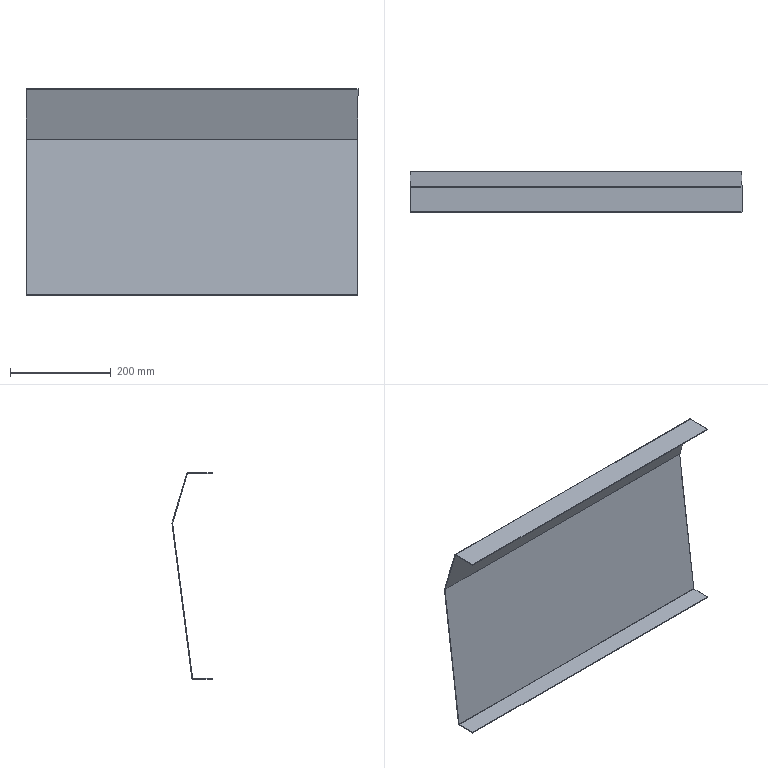Component | SolidWorks | RainproofTopCover-1 | 1 solid | 30 faces | box 660 x 79.97 x 410 mm | volume 498730 mm3 | plane 24 | cylinder 6 | commonest cylinder face diameters 3.2 x3 0.2 x3
STEP:
#1=COLOUR_RGB('',0.7922,0.8196,0.9333);
#2=FILL_AREA_STYLE_COLOUR('',#1);
#3=FILL_AREA_STYLE('',(#2));
#4=SURFACE_STYLE_FILL_AREA(#3);
#5=SURFACE_SIDE_STYLE('',(#4));
#6=SURFACE_STYLE_USAGE(.BOTH.,#5);
#7=PRESENTATION_STYLE_ASSIGNMENT((#6));
#8=CARTESIAN_POINT('',(-14.739,15.415,23.545));
#9=VERTEX_POINT('',#8);
#10=CARTESIAN_POINT('',(-14.739,15.357,23.552));
#11=VERTEX_POINT('',#10);
#12=CARTESIAN_POINT('',(-14.739,15.415,23.545));
#13=DIRECTION('',(0.,-0.9918,0.128));
#14=VECTOR('',#13,39.37);
#15=LINE('',#12,#14);
#16=EDGE_CURVE('',#9,#11,#15,.T.);
#17=ORIENTED_EDGE('',*,*,#16,.F.);
#18=CARTESIAN_POINT('',(-14.739,15.353,23.49));
#19=VERTEX_POINT('',#18);
#20=CARTESIAN_POINT('',(-14.739,15.353,23.553));
#21=DIRECTION('',(1.,0.,-0.));
#22=DIRECTION('',(0.,0.,1.));
#23=AXIS2_PLACEMENT_3D('',#20,#21,#22);
#24=CIRCLE('',#23,0.06299);
#25=EDGE_CURVE('',#19,#9,#24,.T.);
#26=ORIENTED_EDGE('',*,*,#25,.F.);
#27=CARTESIAN_POINT('',(-14.739,15.353,23.549));
#28=VERTEX_POINT('',#27);
#29=CARTESIAN_POINT('',(-14.739,15.353,23.549));
#30=DIRECTION('',(-0.,0.,-1.));
#31=VECTOR('',#30,39.37);
#32=LINE('',#29,#31);
#33=EDGE_CURVE('',#28,#19,#32,.T.);
#34=ORIENTED_EDGE('',*,*,#33,.F.);
#35=CARTESIAN_POINT('',(-14.739,15.353,23.553));
#36=DIRECTION('',(1.,0.,-0.));
#37=DIRECTION('',(0.,0.,1.));
#38=AXIS2_PLACEMENT_3D('',#35,#36,#37);
#39=CIRCLE('',#38,0.003937);
#40=EDGE_CURVE('',#28,#11,#39,.T.);
#41=ORIENTED_EDGE('',*,*,#40,.T.);
#42=EDGE_LOOP('',(#17,#26,#34,#41));
#43=FACE_OUTER_BOUND('',#42,.T.);
#44=CARTESIAN_POINT('',(-14.739,15.415,23.545));
#45=DIRECTION('',(-1.,-0.,0.));
#46=DIRECTION('',(0.,-0.,1.));
#47=AXIS2_PLACEMENT_3D('',#44,#45,#46);
#48=PLANE('',#47);
#49=ADVANCED_FACE('',(#43),#48,.T.);
#50=CARTESIAN_POINT('',(-14.739,16.981,35.681));
#51=VERTEX_POINT('',#50);
#52=CARTESIAN_POINT('',(-14.739,15.408,23.49));
#53=DIRECTION('',(0.,0.128,0.9918));
#54=VECTOR('',#53,39.37);
#55=LINE('',#52,#54);
#56=EDGE_CURVE('',#9,#51,#55,.T.);
#57=ORIENTED_EDGE('',*,*,#56,.F.);
#58=ORIENTED_EDGE('',*,*,#16,.T.);
#59=CARTESIAN_POINT('',(-14.739,16.923,35.689));
#60=VERTEX_POINT('',#59);
#61=CARTESIAN_POINT('',(-14.739,15.35,23.497));
#62=DIRECTION('',(0.,0.128,0.9918));
#63=VECTOR('',#62,39.37);
#64=LINE('',#61,#63);
#65=EDGE_CURVE('',#11,#60,#64,.T.);
#66=ORIENTED_EDGE('',*,*,#65,.T.);
#67=CARTESIAN_POINT('',(-14.739,16.923,35.689));
#68=DIRECTION('',(-0.,0.9918,-0.128));
#69=VECTOR('',#68,39.37);
#70=LINE('',#67,#69);
#71=EDGE_CURVE('',#60,#51,#70,.T.);
#72=ORIENTED_EDGE('',*,*,#71,.T.);
#73=EDGE_LOOP('',(#57,#58,#66,#72));
#74=FACE_OUTER_BOUND('',#73,.T.);
#75=CARTESIAN_POINT('',(-14.739,15.353,23.549));
#76=DIRECTION('',(-1.,-0.,0.));
#77=DIRECTION('',(0.,-0.,1.));
#78=AXIS2_PLACEMENT_3D('',#75,#76,#77);
#79=PLANE('',#78);
#80=ADVANCED_FACE('',(#74),#79,.T.);
#81=CARTESIAN_POINT('',(11.246,15.353,23.49));
#82=VERTEX_POINT('',#81);
#83=CARTESIAN_POINT('',(11.246,15.353,23.549));
#84=VERTEX_POINT('',#83);
#85=CARTESIAN_POINT('',(11.246,15.353,23.49));
#86=DIRECTION('',(0.,-0.,1.));
#87=VECTOR('',#86,39.37);
#88=LINE('',#85,#87);
#89=EDGE_CURVE('',#82,#84,#88,.T.);
#90=ORIENTED_EDGE('',*,*,#89,.F.);
#91=CARTESIAN_POINT('',(11.246,15.415,23.545));
#92=VERTEX_POINT('',#91);
#93=CARTESIAN_POINT('',(11.246,15.353,23.553));
#94=DIRECTION('',(1.,0.,-0.));
#95=DIRECTION('',(0.,0.,1.));
#96=AXIS2_PLACEMENT_3D('',#93,#94,#95);
#97=CIRCLE('',#96,0.06299);
#98=EDGE_CURVE('',#82,#92,#97,.T.);
#99=ORIENTED_EDGE('',*,*,#98,.T.);
#100=CARTESIAN_POINT('',(11.246,15.357,23.552));
#101=VERTEX_POINT('',#100);
#102=CARTESIAN_POINT('',(11.246,15.357,23.552));
#103=DIRECTION('',(-0.,0.9918,-0.128));
#104=VECTOR('',#103,39.37);
#105=LINE('',#102,#104);
#106=EDGE_CURVE('',#101,#92,#105,.T.);
#107=ORIENTED_EDGE('',*,*,#106,.F.);
#108=CARTESIAN_POINT('',(11.246,15.353,23.553));
#109=DIRECTION('',(1.,0.,-0.));
#110=DIRECTION('',(0.,0.,1.));
#111=AXIS2_PLACEMENT_3D('',#108,#109,#110);
#112=CIRCLE('',#111,0.003937);
#113=EDGE_CURVE('',#84,#101,#112,.T.);
#114=ORIENTED_EDGE('',*,*,#113,.F.);
#115=EDGE_LOOP('',(#90,#99,#107,#114));
#116=FACE_OUTER_BOUND('',#115,.T.);
#117=CARTESIAN_POINT('',(11.246,15.353,23.49));
#118=DIRECTION('',(1.,0.,-0.));
#119=DIRECTION('',(-0.,0.,-1.));
#120=AXIS2_PLACEMENT_3D('',#117,#118,#119);
#121=PLANE('',#120);
#122=ADVANCED_FACE('',(#116),#121,.T.);
#123=CARTESIAN_POINT('',(11.246,13.833,23.49));
#124=VERTEX_POINT('',#123);
#125=CARTESIAN_POINT('',(11.246,13.833,23.49));
#126=DIRECTION('',(0.,1.,0.));
#127=VECTOR('',#126,39.37);
#128=LINE('',#125,#127);
#129=EDGE_CURVE('',#124,#82,#128,.T.);
#130=ORIENTED_EDGE('',*,*,#129,.T.);
#131=ORIENTED_EDGE('',*,*,#89,.T.);
#132=CARTESIAN_POINT('',(11.246,13.833,23.549));
#133=VERTEX_POINT('',#132);
#134=CARTESIAN_POINT('',(11.246,13.833,23.549));
#135=DIRECTION('',(0.,1.,0.));
#136=VECTOR('',#135,39.37);
#137=LINE('',#134,#136);
#138=EDGE_CURVE('',#133,#84,#137,.T.);
#139=ORIENTED_EDGE('',*,*,#138,.F.);
#140=CARTESIAN_POINT('',(11.246,13.833,23.549));
#141=DIRECTION('',(-0.,0.,-1.));
#142=VECTOR('',#141,39.37);
#143=LINE('',#140,#142);
#144=EDGE_CURVE('',#133,#124,#143,.T.);
#145=ORIENTED_EDGE('',*,*,#144,.T.);
#146=EDGE_LOOP('',(#130,#131,#139,#145));
#147=FACE_OUTER_BOUND('',#146,.T.);
#148=CARTESIAN_POINT('',(11.246,15.357,23.552));
#149=DIRECTION('',(1.,0.,-0.));
#150=DIRECTION('',(-0.,0.,-1.));
#151=AXIS2_PLACEMENT_3D('',#148,#149,#150);
#152=PLANE('',#151);
#153=ADVANCED_FACE('',(#147),#152,.T.);
#154=CARTESIAN_POINT('',(-14.739,16.979,35.707));
#155=VERTEX_POINT('',#154);
#156=CARTESIAN_POINT('',(-14.739,16.923,35.69));
#157=VERTEX_POINT('',#156);
#158=CARTESIAN_POINT('',(-14.739,16.979,35.707));
#159=DIRECTION('',(-0.,-0.9578,-0.2873));
#160=VECTOR('',#159,39.37);
#161=LINE('',#158,#160);
#162=EDGE_CURVE('',#155,#157,#161,.T.);
#163=ORIENTED_EDGE('',*,*,#162,.F.);
#164=CARTESIAN_POINT('',(-14.739,16.919,35.689));
#165=DIRECTION('',(1.,0.,-0.));
#166=DIRECTION('',(0.,0.,1.));
#167=AXIS2_PLACEMENT_3D('',#164,#165,#166);
#168=CIRCLE('',#167,0.06299);
#169=EDGE_CURVE('',#51,#155,#168,.T.);
#170=ORIENTED_EDGE('',*,*,#169,.F.);
#171=ORIENTED_EDGE('',*,*,#71,.F.);
#172=CARTESIAN_POINT('',(-14.739,16.919,35.689));
#173=DIRECTION('',(1.,0.,-0.));
#174=DIRECTION('',(0.,0.,1.));
#175=AXIS2_PLACEMENT_3D('',#172,#173,#174);
#176=CIRCLE('',#175,0.003937);
#177=EDGE_CURVE('',#60,#157,#176,.T.);
#178=ORIENTED_EDGE('',*,*,#177,.T.);
#179=EDGE_LOOP('',(#163,#170,#171,#178));
#180=FACE_OUTER_BOUND('',#179,.T.);
#181=CARTESIAN_POINT('',(-14.739,16.979,35.707));
#182=DIRECTION('',(-1.,-0.,0.));
#183=DIRECTION('',(0.,-0.,1.));
#184=AXIS2_PLACEMENT_3D('',#181,#182,#183);
#185=PLANE('',#184);
#186=ADVANCED_FACE('',(#180),#185,.T.);
#187=CARTESIAN_POINT('',(-14.739,15.815,39.586));
#188=VERTEX_POINT('',#187);
#189=CARTESIAN_POINT('',(-14.739,16.983,35.694));
#190=DIRECTION('',(0.,-0.2873,0.9578));
#191=VECTOR('',#190,39.37);
#192=LINE('',#189,#191);
#193=EDGE_CURVE('',#155,#188,#192,.T.);
#194=ORIENTED_EDGE('',*,*,#193,.F.);
#195=ORIENTED_EDGE('',*,*,#162,.T.);
#196=CARTESIAN_POINT('',(-14.739,15.759,39.57));
#197=VERTEX_POINT('',#196);
#198=CARTESIAN_POINT('',(-14.739,16.926,35.677));
#199=DIRECTION('',(0.,-0.2873,0.9578));
#200=VECTOR('',#199,39.37);
#201=LINE('',#198,#200);
#202=EDGE_CURVE('',#157,#197,#201,.T.);
#203=ORIENTED_EDGE('',*,*,#202,.T.);
#204=CARTESIAN_POINT('',(-14.739,15.759,39.57));
#205=DIRECTION('',(0.,0.9578,0.2873));
#206=VECTOR('',#205,39.37);
#207=LINE('',#204,#206);
#208=EDGE_CURVE('',#197,#188,#207,.T.);
#209=ORIENTED_EDGE('',*,*,#208,.T.);
#210=EDGE_LOOP('',(#194,#195,#203,#209));
#211=FACE_OUTER_BOUND('',#210,.T.);
#212=CARTESIAN_POINT('',(-14.739,16.923,35.689));
#213=DIRECTION('',(-1.,-0.,0.));
#214=DIRECTION('',(0.,-0.,1.));
#215=AXIS2_PLACEMENT_3D('',#212,#213,#214);
#216=PLANE('',#215);
#217=ADVANCED_FACE('',(#211),#216,.T.);
#218=CARTESIAN_POINT('',(11.246,16.981,35.681));
#219=VERTEX_POINT('',#218);
#220=CARTESIAN_POINT('',(11.246,16.923,35.689));
#221=VERTEX_POINT('',#220);
#222=CARTESIAN_POINT('',(11.246,16.981,35.681));
#223=DIRECTION('',(0.,-0.9918,0.128));
#224=VECTOR('',#223,39.37);
#225=LINE('',#222,#224);
#226=EDGE_CURVE('',#219,#221,#225,.T.);
#227=ORIENTED_EDGE('',*,*,#226,.F.);
#228=CARTESIAN_POINT('',(11.246,16.979,35.707));
#229=VERTEX_POINT('',#228);
#230=CARTESIAN_POINT('',(11.246,16.919,35.689));
#231=DIRECTION('',(1.,0.,-0.));
#232=DIRECTION('',(0.,0.,1.));
#233=AXIS2_PLACEMENT_3D('',#230,#231,#232);
#234=CIRCLE('',#233,0.06299);
#235=EDGE_CURVE('',#219,#229,#234,.T.);
#236=ORIENTED_EDGE('',*,*,#235,.T.);
#237=CARTESIAN_POINT('',(11.246,16.923,35.69));
#238=VERTEX_POINT('',#237);
#239=CARTESIAN_POINT('',(11.246,16.923,35.69));
#240=DIRECTION('',(0.,0.9578,0.2873));
#241=VECTOR('',#240,39.37);
#242=LINE('',#239,#241);
#243=EDGE_CURVE('',#238,#229,#242,.T.);
#244=ORIENTED_EDGE('',*,*,#243,.F.);
#245=CARTESIAN_POINT('',(11.246,16.919,35.689));
#246=DIRECTION('',(1.,0.,-0.));
#247=DIRECTION('',(0.,0.,1.));
#248=AXIS2_PLACEMENT_3D('',#245,#246,#247);
#249=CIRCLE('',#248,0.003937);
#250=EDGE_CURVE('',#221,#238,#249,.T.);
#251=ORIENTED_EDGE('',*,*,#250,.F.);
#252=EDGE_LOOP('',(#227,#236,#244,#251));
#253=FACE_OUTER_BOUND('',#252,.T.);
#254=CARTESIAN_POINT('',(11.246,16.981,35.681));
#255=DIRECTION('',(1.,0.,-0.));
#256=DIRECTION('',(-0.,0.,-1.));
#257=AXIS2_PLACEMENT_3D('',#254,#255,#256);
#258=PLANE('',#257);
#259=ADVANCED_FACE('',(#253),#258,.T.);
#260=CARTESIAN_POINT('',(11.246,15.408,23.49));
#261=DIRECTION('',(0.,0.128,0.9918));
#262=VECTOR('',#261,39.37);
#263=LINE('',#260,#262);
#264=EDGE_CURVE('',#92,#219,#263,.T.);
#265=ORIENTED_EDGE('',*,*,#264,.T.);
#266=ORIENTED_EDGE('',*,*,#226,.T.);
#267=CARTESIAN_POINT('',(11.246,15.35,23.497));
#268=DIRECTION('',(0.,0.128,0.9918));
#269=VECTOR('',#268,39.37);
#270=LINE('',#267,#269);
#271=EDGE_CURVE('',#101,#221,#270,.T.);
#272=ORIENTED_EDGE('',*,*,#271,.F.);
#273=ORIENTED_EDGE('',*,*,#106,.T.);
#274=EDGE_LOOP('',(#265,#266,#272,#273));
#275=FACE_OUTER_BOUND('',#274,.T.);
#276=CARTESIAN_POINT('',(11.246,16.923,35.69));
#277=DIRECTION('',(1.,0.,-0.));
#278=DIRECTION('',(-0.,0.,-1.));
#279=AXIS2_PLACEMENT_3D('',#276,#277,#278);
#280=PLANE('',#279);
#281=ADVANCED_FACE('',(#275),#280,.T.);
#282=CARTESIAN_POINT('',(-14.739,15.755,39.631));
#283=VERTEX_POINT('',#282);
#284=CARTESIAN_POINT('',(-14.739,15.755,39.572));
#285=VERTEX_POINT('',#284);
#286=CARTESIAN_POINT('',(-14.739,15.755,39.631));
#287=DIRECTION('',(-0.,0.,-1.));
#288=VECTOR('',#287,39.37);
#289=LINE('',#286,#288);
#290=EDGE_CURVE('',#283,#285,#289,.T.);
#291=ORIENTED_EDGE('',*,*,#290,.F.);
#292=CARTESIAN_POINT('',(-14.739,15.755,39.568));
#293=DIRECTION('',(1.,0.,-0.));
#294=DIRECTION('',(0.,-0.,1.));
#295=AXIS2_PLACEMENT_3D('',#292,#293,#294);
#296=CIRCLE('',#295,0.06299);
#297=EDGE_CURVE('',#188,#283,#296,.T.);
#298=ORIENTED_EDGE('',*,*,#297,.F.);
#299=ORIENTED_EDGE('',*,*,#208,.F.);
#300=CARTESIAN_POINT('',(-14.739,15.755,39.568));
#301=DIRECTION('',(1.,0.,-0.));
#302=DIRECTION('',(0.,0.,1.));
#303=AXIS2_PLACEMENT_3D('',#300,#301,#302);
#304=CIRCLE('',#303,0.003937);
#305=EDGE_CURVE('',#197,#285,#304,.T.);
#306=ORIENTED_EDGE('',*,*,#305,.T.);
#307=EDGE_LOOP('',(#291,#298,#299,#306));
#308=FACE_OUTER_BOUND('',#307,.T.);
#309=CARTESIAN_POINT('',(-14.739,15.755,39.631));
#310=DIRECTION('',(-1.,-0.,0.));
#311=DIRECTION('',(0.,-0.,1.));
#312=AXIS2_PLACEMENT_3D('',#309,#310,#311);
#313=PLANE('',#312);
#314=ADVANCED_FACE('',(#308),#313,.T.);
#315=CARTESIAN_POINT('',(-14.739,13.833,39.631));
#316=VERTEX_POINT('',#315);
#317=CARTESIAN_POINT('',(-14.739,15.802,39.631));
#318=DIRECTION('',(0.,-1.,-0.));
#319=VECTOR('',#318,39.37);
#320=LINE('',#317,#319);
#321=EDGE_CURVE('',#283,#316,#320,.T.);
#322=ORIENTED_EDGE('',*,*,#321,.F.);
#323=ORIENTED_EDGE('',*,*,#290,.T.);
#324=CARTESIAN_POINT('',(-14.739,13.833,39.572));
#325=VERTEX_POINT('',#324);
#326=CARTESIAN_POINT('',(-14.739,15.802,39.572));
#327=DIRECTION('',(0.,-1.,-0.));
#328=VECTOR('',#327,39.37);
#329=LINE('',#326,#328);
#330=EDGE_CURVE('',#285,#325,#329,.T.);
#331=ORIENTED_EDGE('',*,*,#330,.T.);
#332=CARTESIAN_POINT('',(-14.739,13.833,39.631));
#333=DIRECTION('',(-0.,0.,-1.));
#334=VECTOR('',#333,39.37);
#335=LINE('',#332,#334);
#336=EDGE_CURVE('',#316,#325,#335,.T.);
#337=ORIENTED_EDGE('',*,*,#336,.F.);
#338=EDGE_LOOP('',(#322,#323,#331,#337));
#339=FACE_OUTER_BOUND('',#338,.T.);
#340=CARTESIAN_POINT('',(-14.739,15.759,39.57));
#341=DIRECTION('',(-1.,-0.,0.));
#342=DIRECTION('',(0.,-0.,1.));
#343=AXIS2_PLACEMENT_3D('',#340,#341,#342);
#344=PLANE('',#343);
#345=ADVANCED_FACE('',(#339),#344,.T.);
#346=CARTESIAN_POINT('',(11.246,15.815,39.586));
#347=VERTEX_POINT('',#346);
#348=CARTESIAN_POINT('',(11.246,15.759,39.57));
#349=VERTEX_POINT('',#348);
#350=CARTESIAN_POINT('',(11.246,15.815,39.586));
#351=DIRECTION('',(-0.,-0.9578,-0.2873));
#352=VECTOR('',#351,39.37);
#353=LINE('',#350,#352);
#354=EDGE_CURVE('',#347,#349,#353,.T.);
#355=ORIENTED_EDGE('',*,*,#354,.F.);
#356=CARTESIAN_POINT('',(11.246,15.755,39.631));
#357=VERTEX_POINT('',#356);
#358=CARTESIAN_POINT('',(11.246,15.755,39.568));
#359=DIRECTION('',(1.,0.,-0.));
#360=DIRECTION('',(0.,0.,1.));
#361=AXIS2_PLACEMENT_3D('',#358,#359,#360);
#362=CIRCLE('',#361,0.06299);
#363=EDGE_CURVE('',#347,#357,#362,.T.);
#364=ORIENTED_EDGE('',*,*,#363,.T.);
#365=CARTESIAN_POINT('',(11.246,15.755,39.572));
#366=VERTEX_POINT('',#365);
#367=CARTESIAN_POINT('',(11.246,15.755,39.572));
#368=DIRECTION('',(0.,-0.,1.));
#369=VECTOR('',#368,39.37);
#370=LINE('',#367,#369);
#371=EDGE_CURVE('',#366,#357,#370,.T.);
#372=ORIENTED_EDGE('',*,*,#371,.F.);
#373=CARTESIAN_POINT('',(11.246,15.755,39.568));
#374=DIRECTION('',(1.,0.,-0.));
#375=DIRECTION('',(0.,0.,1.));
#376=AXIS2_PLACEMENT_3D('',#373,#374,#375);
#377=CIRCLE('',#376,0.003937);
#378=EDGE_CURVE('',#349,#366,#377,.T.);
#379=ORIENTED_EDGE('',*,*,#378,.F.);
#380=EDGE_LOOP('',(#355,#364,#372,#379));
#381=FACE_OUTER_BOUND('',#380,.T.);
#382=CARTESIAN_POINT('',(11.246,15.815,39.586));
#383=DIRECTION('',(1.,0.,-0.));
#384=DIRECTION('',(-0.,0.,-1.));
#385=AXIS2_PLACEMENT_3D('',#382,#383,#384);
#386=PLANE('',#385);
#387=ADVANCED_FACE('',(#381),#386,.T.);
#388=CARTESIAN_POINT('',(11.246,16.983,35.694));
#389=DIRECTION('',(0.,-0.2873,0.9578));
#390=VECTOR('',#389,39.37);
#391=LINE('',#388,#390);
#392=EDGE_CURVE('',#229,#347,#391,.T.);
#393=ORIENTED_EDGE('',*,*,#392,.T.);
#394=ORIENTED_EDGE('',*,*,#354,.T.);
#395=CARTESIAN_POINT('',(11.246,16.926,35.677));
#396=DIRECTION('',(0.,-0.2873,0.9578));
#397=VECTOR('',#396,39.37);
#398=LINE('',#395,#397);
#399=EDGE_CURVE('',#238,#349,#398,.T.);
#400=ORIENTED_EDGE('',*,*,#399,.F.);
#401=ORIENTED_EDGE('',*,*,#243,.T.);
#402=EDGE_LOOP('',(#393,#394,#400,#401));
#403=FACE_OUTER_BOUND('',#402,.T.);
#404=CARTESIAN_POINT('',(11.246,15.755,39.572));
#405=DIRECTION('',(1.,0.,-0.));
#406=DIRECTION('',(-0.,0.,-1.));
#407=AXIS2_PLACEMENT_3D('',#404,#405,#406);
#408=PLANE('',#407);
#409=ADVANCED_FACE('',(#403),#408,.T.);
#410=CARTESIAN_POINT('',(11.246,13.833,39.572));
#411=VERTEX_POINT('',#410);
#412=CARTESIAN_POINT('',(11.246,15.802,39.572));
#413=DIRECTION('',(0.,-1.,-0.));
#414=VECTOR('',#413,39.37);
#415=LINE('',#412,#414);
#416=EDGE_CURVE('',#366,#411,#415,.T.);
#417=ORIENTED_EDGE('',*,*,#416,.T.);
#418=CARTESIAN_POINT('',(-14.739,13.833,39.572));
#419=DIRECTION('',(1.,0.,-0.));
#420=VECTOR('',#419,39.37);
#421=LINE('',#418,#420);
#422=EDGE_CURVE('',#325,#411,#421,.T.);
#423=ORIENTED_EDGE('',*,*,#422,.F.);
#424=ORIENTED_EDGE('',*,*,#330,.F.);
#425=CARTESIAN_POINT('',(-14.739,15.755,39.572));
#426=DIRECTION('',(1.,0.,-0.));
#427=VECTOR('',#426,39.37);
#428=LINE('',#425,#427);
#429=EDGE_CURVE('',#285,#366,#428,.T.);
#430=ORIENTED_EDGE('',*,*,#429,.T.);
#431=EDGE_LOOP('',(#417,#423,#424,#430));
#432=FACE_OUTER_BOUND('',#431,.T.);
#433=CARTESIAN_POINT('',(-14.739,15.802,39.572));
#434=DIRECTION('',(0.,-0.,1.));
#435=DIRECTION('',(1.,0.,-0.));
#436=AXIS2_PLACEMENT_3D('',#433,#434,#435);
#437=PLANE('',#436);
#438=ADVANCED_FACE('',(#432),#437,.F.);
#439=CARTESIAN_POINT('',(11.246,13.833,39.631));
#440=VERTEX_POINT('',#439);
#441=CARTESIAN_POINT('',(11.246,13.833,39.631));
#442=DIRECTION('',(-0.,0.,-1.));
#443=VECTOR('',#442,39.37);
#444=LINE('',#441,#443);
#445=EDGE_CURVE('',#440,#411,#444,.T.);
#446=ORIENTED_EDGE('',*,*,#445,.F.);
#447=CARTESIAN_POINT('',(-14.739,13.833,39.631));
#448=DIRECTION('',(1.,0.,-0.));
#449=VECTOR('',#448,39.37);
#450=LINE('',#447,#449);
#451=EDGE_CURVE('',#316,#440,#450,.T.);
#452=ORIENTED_EDGE('',*,*,#451,.F.);
#453=ORIENTED_EDGE('',*,*,#336,.T.);
#454=ORIENTED_EDGE('',*,*,#422,.T.);
#455=EDGE_LOOP('',(#446,#452,#453,#454));
#456=FACE_OUTER_BOUND('',#455,.T.);
#457=CARTESIAN_POINT('',(-14.739,13.833,39.631));
#458=DIRECTION('',(-0.,-1.,-0.));
#459=DIRECTION('',(0.,-0.,1.));
#460=AXIS2_PLACEMENT_3D('',#457,#458,#459);
#461=PLANE('',#460);
#462=ADVANCED_FACE('',(#456),#461,.T.);
#463=CARTESIAN_POINT('',(11.246,15.802,39.631));
#464=DIRECTION('',(0.,-1.,-0.));
#465=VECTOR('',#464,39.37);
#466=LINE('',#463,#465);
#467=EDGE_CURVE('',#357,#440,#466,.T.);
#468=ORIENTED_EDGE('',*,*,#467,.F.);
#469=CARTESIAN_POINT('',(-14.739,15.755,39.631));
#470=DIRECTION('',(1.,0.,-0.));
#471=VECTOR('',#470,39.37);
#472=LINE('',#469,#471);
#473=EDGE_CURVE('',#283,#357,#472,.T.);
#474=ORIENTED_EDGE('',*,*,#473,.F.);
#475=ORIENTED_EDGE('',*,*,#321,.T.);
#476=ORIENTED_EDGE('',*,*,#451,.T.);
#477=EDGE_LOOP('',(#468,#474,#475,#476));
#478=FACE_OUTER_BOUND('',#477,.T.);
#479=CARTESIAN_POINT('',(-14.739,15.802,39.631));
#480=DIRECTION('',(0.,-0.,1.));
#481=DIRECTION('',(1.,0.,-0.));
#482=AXIS2_PLACEMENT_3D('',#479,#480,#481);
#483=PLANE('',#482);
#484=ADVANCED_FACE('',(#478),#483,.T.);
#485=ORIENTED_EDGE('',*,*,#363,.F.);
#486=CARTESIAN_POINT('',(-14.739,15.815,39.586));
#487=DIRECTION('',(1.,0.,-0.));
#488=VECTOR('',#487,39.37);
#489=LINE('',#486,#488);
#490=EDGE_CURVE('',#188,#347,#489,.T.);
#491=ORIENTED_EDGE('',*,*,#490,.F.);
#492=ORIENTED_EDGE('',*,*,#297,.T.);
#493=ORIENTED_EDGE('',*,*,#473,.T.);
#494=EDGE_LOOP('',(#485,#491,#492,#493));
#495=FACE_OUTER_BOUND('',#494,.T.);
#496=CARTESIAN_POINT('',(-14.739,15.755,39.568));
#497=DIRECTION('',(1.,0.,-0.));
#498=DIRECTION('',(0.,0.,-1.));
#499=AXIS2_PLACEMENT_3D('',#496,#497,#498);
#500=CYLINDRICAL_SURFACE('',#499,0.06299);
#501=ADVANCED_FACE('',(#495),#500,.T.);
#502=ORIENTED_EDGE('',*,*,#392,.F.);
#503=CARTESIAN_POINT('',(-14.739,16.979,35.707));
#504=DIRECTION('',(1.,0.,-0.));
#505=VECTOR('',#504,39.37);
#506=LINE('',#503,#505);
#507=EDGE_CURVE('',#155,#229,#506,.T.);
#508=ORIENTED_EDGE('',*,*,#507,.F.);
#509=ORIENTED_EDGE('',*,*,#193,.T.);
#510=ORIENTED_EDGE('',*,*,#490,.T.);
#511=EDGE_LOOP('',(#502,#508,#509,#510));
#512=FACE_OUTER_BOUND('',#511,.T.);
#513=CARTESIAN_POINT('',(-14.739,16.983,35.694));
#514=DIRECTION('',(0.,0.9578,0.2873));
#515=DIRECTION('',(-0.,0.2873,-0.9578));
#516=AXIS2_PLACEMENT_3D('',#513,#514,#515);
#517=PLANE('',#516);
#518=ADVANCED_FACE('',(#512),#517,.T.);
#519=ORIENTED_EDGE('',*,*,#235,.F.);
#520=CARTESIAN_POINT('',(-14.739,16.981,35.681));
#521=DIRECTION('',(1.,0.,-0.));
#522=VECTOR('',#521,39.37);
#523=LINE('',#520,#522);
#524=EDGE_CURVE('',#51,#219,#523,.T.);
#525=ORIENTED_EDGE('',*,*,#524,.F.);
#526=ORIENTED_EDGE('',*,*,#169,.T.);
#527=ORIENTED_EDGE('',*,*,#507,.T.);
#528=EDGE_LOOP('',(#519,#525,#526,#527));
#529=FACE_OUTER_BOUND('',#528,.T.);
#530=CARTESIAN_POINT('',(-14.739,16.919,35.689));
#531=DIRECTION('',(1.,0.,-0.));
#532=DIRECTION('',(0.,0.,-1.));
#533=AXIS2_PLACEMENT_3D('',#530,#531,#532);
#534=CYLINDRICAL_SURFACE('',#533,0.06299);
#535=ADVANCED_FACE('',(#529),#534,.T.);
#536=ORIENTED_EDGE('',*,*,#264,.F.);
#537=CARTESIAN_POINT('',(-14.739,15.415,23.545));
#538=DIRECTION('',(1.,0.,-0.));
#539=VECTOR('',#538,39.37);
#540=LINE('',#537,#539);
#541=EDGE_CURVE('',#9,#92,#540,.T.);
#542=ORIENTED_EDGE('',*,*,#541,.F.);
#543=ORIENTED_EDGE('',*,*,#56,.T.);
#544=ORIENTED_EDGE('',*,*,#524,.T.);
#545=EDGE_LOOP('',(#536,#542,#543,#544));
#546=FACE_OUTER_BOUND('',#545,.T.);
#547=CARTESIAN_POINT('',(-14.739,15.408,23.49));
#548=DIRECTION('',(-0.,0.9918,-0.128));
#549=DIRECTION('',(-0.,-0.128,-0.9918));
#550=AXIS2_PLACEMENT_3D('',#547,#548,#549);
#551=PLANE('',#550);
#552=ADVANCED_FACE('',(#546),#551,.T.);
#553=ORIENTED_EDGE('',*,*,#98,.F.);
#554=CARTESIAN_POINT('',(-14.739,15.353,23.49));
#555=DIRECTION('',(1.,0.,-0.));
#556=VECTOR('',#555,39.37);
#557=LINE('',#554,#556);
#558=EDGE_CURVE('',#19,#82,#557,.T.);
#559=ORIENTED_EDGE('',*,*,#558,.F.);
#560=ORIENTED_EDGE('',*,*,#25,.T.);
#561=ORIENTED_EDGE('',*,*,#541,.T.);
#562=EDGE_LOOP('',(#553,#559,#560,#561));
#563=FACE_OUTER_BOUND('',#562,.T.);
#564=CARTESIAN_POINT('',(-14.739,15.353,23.553));
#565=DIRECTION('',(1.,0.,-0.));
#566=DIRECTION('',(0.,0.,-1.));
#567=AXIS2_PLACEMENT_3D('',#564,#565,#566);
#568=CYLINDRICAL_SURFACE('',#567,0.06299);
#569=ADVANCED_FACE('',(#563),#568,.T.);
#570=ORIENTED_EDGE('',*,*,#129,.F.);
#571=CARTESIAN_POINT('',(-14.739,13.833,23.49));
#572=VERTEX_POINT('',#571);
#573=CARTESIAN_POINT('',(-14.739,13.833,23.49));
#574=DIRECTION('',(1.,0.,-0.));
#575=VECTOR('',#574,39.37);
#576=LINE('',#573,#575);
#577=EDGE_CURVE('',#572,#124,#576,.T.);
#578=ORIENTED_EDGE('',*,*,#577,.F.);
#579=CARTESIAN_POINT('',(-14.739,13.833,23.49));
#580=DIRECTION('',(0.,1.,0.));
#581=VECTOR('',#580,39.37);
#582=LINE('',#579,#581);
#583=EDGE_CURVE('',#572,#19,#582,.T.);
#584=ORIENTED_EDGE('',*,*,#583,.T.);
#585=ORIENTED_EDGE('',*,*,#558,.T.);
#586=EDGE_LOOP('',(#570,#578,#584,#585));
#587=FACE_OUTER_BOUND('',#586,.T.);
#588=CARTESIAN_POINT('',(-14.739,13.833,23.49));
#589=DIRECTION('',(-0.,0.,-1.));
#590=DIRECTION('',(-1.,0.,0.));
#591=AXIS2_PLACEMENT_3D('',#588,#589,#590);
#592=PLANE('',#591);
#593=ADVANCED_FACE('',(#587),#592,.T.);
#594=ORIENTED_EDGE('',*,*,#144,.F.);
#595=CARTESIAN_POINT('',(-14.739,13.833,23.549));
#596=VERTEX_POINT('',#595);
#597=CARTESIAN_POINT('',(-14.739,13.833,23.549));
#598=DIRECTION('',(1.,0.,-0.));
#599=VECTOR('',#598,39.37);
#600=LINE('',#597,#599);
#601=EDGE_CURVE('',#596,#133,#600,.T.);
#602=ORIENTED_EDGE('',*,*,#601,.F.);
#603=CARTESIAN_POINT('',(-14.739,13.833,23.549));
#604=DIRECTION('',(-0.,0.,-1.));
#605=VECTOR('',#604,39.37);
#606=LINE('',#603,#605);
#607=EDGE_CURVE('',#596,#572,#606,.T.);
#608=ORIENTED_EDGE('',*,*,#607,.T.);
#609=ORIENTED_EDGE('',*,*,#577,.T.);
#610=EDGE_LOOP('',(#594,#602,#608,#609));
#611=FACE_OUTER_BOUND('',#610,.T.);
#612=CARTESIAN_POINT('',(-14.739,13.833,23.549));
#613=DIRECTION('',(-0.,-1.,-0.));
#614=DIRECTION('',(0.,-0.,1.));
#615=AXIS2_PLACEMENT_3D('',#612,#613,#614);
#616=PLANE('',#615);
#617=ADVANCED_FACE('',(#611),#616,.T.);
#618=ORIENTED_EDGE('',*,*,#138,.T.);
#619=CARTESIAN_POINT('',(-14.739,15.353,23.549));
#620=DIRECTION('',(1.,0.,-0.));
#621=VECTOR('',#620,39.37);
#622=LINE('',#619,#621);
#623=EDGE_CURVE('',#28,#84,#622,.T.);
#624=ORIENTED_EDGE('',*,*,#623,.F.);
#625=CARTESIAN_POINT('',(-14.739,13.833,23.549));
#626=DIRECTION('',(0.,1.,0.));
#627=VECTOR('',#626,39.37);
#628=LINE('',#625,#627);
#629=EDGE_CURVE('',#596,#28,#628,.T.);
#630=ORIENTED_EDGE('',*,*,#629,.F.);
#631=ORIENTED_EDGE('',*,*,#601,.T.);
#632=EDGE_LOOP('',(#618,#624,#630,#631));
#633=FACE_OUTER_BOUND('',#632,.T.);
#634=CARTESIAN_POINT('',(-14.739,13.833,23.549));
#635=DIRECTION('',(-0.,0.,-1.));
#636=DIRECTION('',(-1.,0.,0.));
#637=AXIS2_PLACEMENT_3D('',#634,#635,#636);
#638=PLANE('',#637);
#639=ADVANCED_FACE('',(#633),#638,.F.);
#640=ORIENTED_EDGE('',*,*,#113,.T.);
#641=CARTESIAN_POINT('',(-14.739,15.357,23.552));
#642=DIRECTION('',(1.,0.,-0.));
#643=VECTOR('',#642,39.37);
#644=LINE('',#641,#643);
#645=EDGE_CURVE('',#11,#101,#644,.T.);
#646=ORIENTED_EDGE('',*,*,#645,.F.);
#647=ORIENTED_EDGE('',*,*,#40,.F.);
#648=ORIENTED_EDGE('',*,*,#623,.T.);
#649=EDGE_LOOP('',(#640,#646,#647,#648));
#650=FACE_OUTER_BOUND('',#649,.T.);
#651=CARTESIAN_POINT('',(-14.739,15.353,23.553));
#652=DIRECTION('',(1.,0.,-0.));
#653=DIRECTION('',(0.,0.,-1.));
#654=AXIS2_PLACEMENT_3D('',#651,#652,#653);
#655=CYLINDRICAL_SURFACE('',#654,0.003937);
#656=ADVANCED_FACE('',(#650),#655,.F.);
#657=ORIENTED_EDGE('',*,*,#271,.T.);
#658=CARTESIAN_POINT('',(-14.739,16.923,35.689));
#659=DIRECTION('',(1.,0.,-0.));
#660=VECTOR('',#659,39.37);
#661=LINE('',#658,#660);
#662=EDGE_CURVE('',#60,#221,#661,.T.);
#663=ORIENTED_EDGE('',*,*,#662,.F.);
#664=ORIENTED_EDGE('',*,*,#65,.F.);
#665=ORIENTED_EDGE('',*,*,#645,.T.);
#666=EDGE_LOOP('',(#657,#663,#664,#665));
#667=FACE_OUTER_BOUND('',#666,.T.);
#668=CARTESIAN_POINT('',(-14.739,15.35,23.497));
#669=DIRECTION('',(-0.,0.9918,-0.128));
#670=DIRECTION('',(-0.,-0.128,-0.9918));
#671=AXIS2_PLACEMENT_3D('',#668,#669,#670);
#672=PLANE('',#671);
#673=ADVANCED_FACE('',(#667),#672,.F.);
#674=ORIENTED_EDGE('',*,*,#250,.T.);
#675=CARTESIAN_POINT('',(-14.739,16.923,35.69));
#676=DIRECTION('',(1.,0.,-0.));
#677=VECTOR('',#676,39.37);
#678=LINE('',#675,#677);
#679=EDGE_CURVE('',#157,#238,#678,.T.);
#680=ORIENTED_EDGE('',*,*,#679,.F.);
#681=ORIENTED_EDGE('',*,*,#177,.F.);
#682=ORIENTED_EDGE('',*,*,#662,.T.);
#683=EDGE_LOOP('',(#674,#680,#681,#682));
#684=FACE_OUTER_BOUND('',#683,.T.);
#685=CARTESIAN_POINT('',(-14.739,16.919,35.689));
#686=DIRECTION('',(1.,0.,-0.));
#687=DIRECTION('',(0.,0.,-1.));
#688=AXIS2_PLACEMENT_3D('',#685,#686,#687);
#689=CYLINDRICAL_SURFACE('',#688,0.003937);
#690=ADVANCED_FACE('',(#684),#689,.F.);
#691=ORIENTED_EDGE('',*,*,#399,.T.);
#692=CARTESIAN_POINT('',(-14.739,15.759,39.57));
#693=DIRECTION('',(1.,0.,-0.));
#694=VECTOR('',#693,39.37);
#695=LINE('',#692,#694);
#696=EDGE_CURVE('',#197,#349,#695,.T.);
#697=ORIENTED_EDGE('',*,*,#696,.F.);
#698=ORIENTED_EDGE('',*,*,#202,.F.);
#699=ORIENTED_EDGE('',*,*,#679,.T.);
#700=EDGE_LOOP('',(#691,#697,#698,#699));
#701=FACE_OUTER_BOUND('',#700,.T.);
#702=CARTESIAN_POINT('',(-14.739,16.926,35.677));
#703=DIRECTION('',(0.,0.9578,0.2873));
#704=DIRECTION('',(-0.,0.2873,-0.9578));
#705=AXIS2_PLACEMENT_3D('',#702,#703,#704);
#706=PLANE('',#705);
#707=ADVANCED_FACE('',(#701),#706,.F.);
#708=ORIENTED_EDGE('',*,*,#378,.T.);
#709=ORIENTED_EDGE('',*,*,#429,.F.);
#710=ORIENTED_EDGE('',*,*,#305,.F.);
#711=ORIENTED_EDGE('',*,*,#696,.T.);
#712=EDGE_LOOP('',(#708,#709,#710,#711));
#713=FACE_OUTER_BOUND('',#712,.T.);
#714=CARTESIAN_POINT('',(-14.739,15.755,39.568));
#715=DIRECTION('',(1.,0.,-0.));
#716=DIRECTION('',(0.,0.,-1.));
#717=AXIS2_PLACEMENT_3D('',#714,#715,#716);
#718=CYLINDRICAL_SURFACE('',#717,0.003937);
#719=ADVANCED_FACE('',(#713),#718,.F.);
#720=ORIENTED_EDGE('',*,*,#629,.T.);
#721=ORIENTED_EDGE('',*,*,#33,.T.);
#722=ORIENTED_EDGE('',*,*,#583,.F.);
#723=ORIENTED_EDGE('',*,*,#607,.F.);
#724=EDGE_LOOP('',(#720,#721,#722,#723));
#725=FACE_OUTER_BOUND('',#724,.T.);
#726=CARTESIAN_POINT('',(-14.739,15.755,39.568));
#727=DIRECTION('',(-1.,-0.,0.));
#728=DIRECTION('',(0.,-0.,1.));
#729=AXIS2_PLACEMENT_3D('',#726,#727,#728);
#730=PLANE('',#729);
#731=ADVANCED_FACE('',(#725),#730,.T.);
#732=ORIENTED_EDGE('',*,*,#416,.F.);
#733=ORIENTED_EDGE('',*,*,#371,.T.);
#734=ORIENTED_EDGE('',*,*,#467,.T.);
#735=ORIENTED_EDGE('',*,*,#445,.T.);
#736=EDGE_LOOP('',(#732,#733,#734,#735));
#737=FACE_OUTER_BOUND('',#736,.T.);
#738=CARTESIAN_POINT('',(11.246,15.755,39.568));
#739=DIRECTION('',(-1.,-0.,0.));
#740=DIRECTION('',(0.,-0.,1.));
#741=AXIS2_PLACEMENT_3D('',#738,#739,#740);
#742=PLANE('',#741);
#743=ADVANCED_FACE('',(#737),#742,.F.);
#744=CLOSED_SHELL('',(#49,#80,#122,#153,#186,#217,#259,#281,#314,#345,#387,#409,#438,#462,#484,#501,#518,#535,#552,#569,#593,#617,#639,#656,#673,#690,#707,#719,#731,#743));
#745=MANIFOLD_SOLID_BREP('',#744);
#746=STYLED_ITEM('',(#7),#745);
#747=(LENGTH_UNIT()NAMED_UNIT(*)SI_UNIT($,.METRE.));
#748=LENGTH_MEASURE_WITH_UNIT(LENGTH_MEASURE(0.0254),#747);
#749=DIMENSIONAL_EXPONENTS(1.,0.,0.,0.,0.,0.,0.);
#750=(CONVERSION_BASED_UNIT('',#748)LENGTH_UNIT()NAMED_UNIT(#749));
#751=UNCERTAINTY_MEASURE_WITH_UNIT(LENGTH_MEASURE(0.00001),#750,'','');
#752=(NAMED_UNIT(*)PLANE_ANGLE_UNIT()SI_UNIT($,.RADIAN.));
#753=(NAMED_UNIT(*)SI_UNIT($,.STERADIAN.)SOLID_ANGLE_UNIT());
#754=(GEOMETRIC_REPRESENTATION_CONTEXT(3)GLOBAL_UNCERTAINTY_ASSIGNED_CONTEXT((#751))GLOBAL_UNIT_ASSIGNED_CONTEXT((#750,#752,#753))REPRESENTATION_CONTEXT('',''));
#755=MECHANICAL_DESIGN_GEOMETRIC_PRESENTATION_REPRESENTATION('',(#746),#754);
#756=PRESENTATION_LAYER_ASSIGNMENT('','',(#746));
#757=CARTESIAN_POINT('',(0.,0.,0.));
#758=DIRECTION('',(0.,0.,1.));
#759=DIRECTION('',(1.,0.,0.));
#760=AXIS2_PLACEMENT_3D('',#757,#758,#759);
#761=(LENGTH_UNIT()NAMED_UNIT(*)SI_UNIT($,.METRE.));
#762=LENGTH_MEASURE_WITH_UNIT(LENGTH_MEASURE(0.0254),#761);
#763=DIMENSIONAL_EXPONENTS(1.,0.,0.,0.,0.,0.,0.);
#764=(CONVERSION_BASED_UNIT('',#762)LENGTH_UNIT()NAMED_UNIT(#763));
#765=UNCERTAINTY_MEASURE_WITH_UNIT(LENGTH_MEASURE(0.00001),#764,'','');
#766=(NAMED_UNIT(*)PLANE_ANGLE_UNIT()SI_UNIT($,.RADIAN.));
#767=(NAMED_UNIT(*)SI_UNIT($,.STERADIAN.)SOLID_ANGLE_UNIT());
#768=(GEOMETRIC_REPRESENTATION_CONTEXT(3)GLOBAL_UNCERTAINTY_ASSIGNED_CONTEXT((#765))GLOBAL_UNIT_ASSIGNED_CONTEXT((#764,#766,#767))REPRESENTATION_CONTEXT('',''));
#769=ADVANCED_BREP_SHAPE_REPRESENTATION('',(#745,#760),#768);